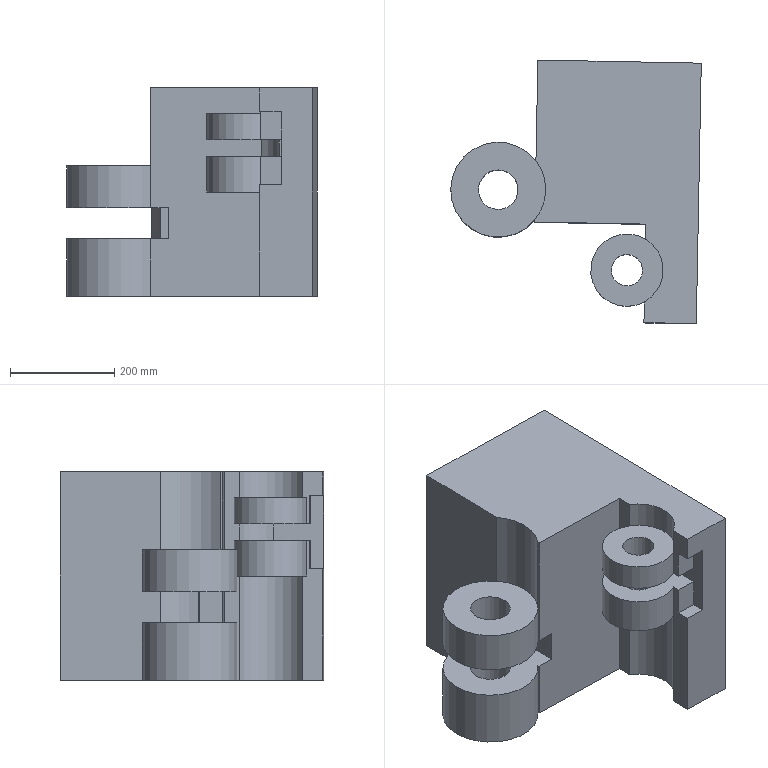Component | NX | FRAME | 1 solid | 40 faces | volume 50102315 mm3 | plane 27 | cylinder 13 | commonest cylinder face diameters 138.98 x5 182.323 x4 60 x2 76 x2